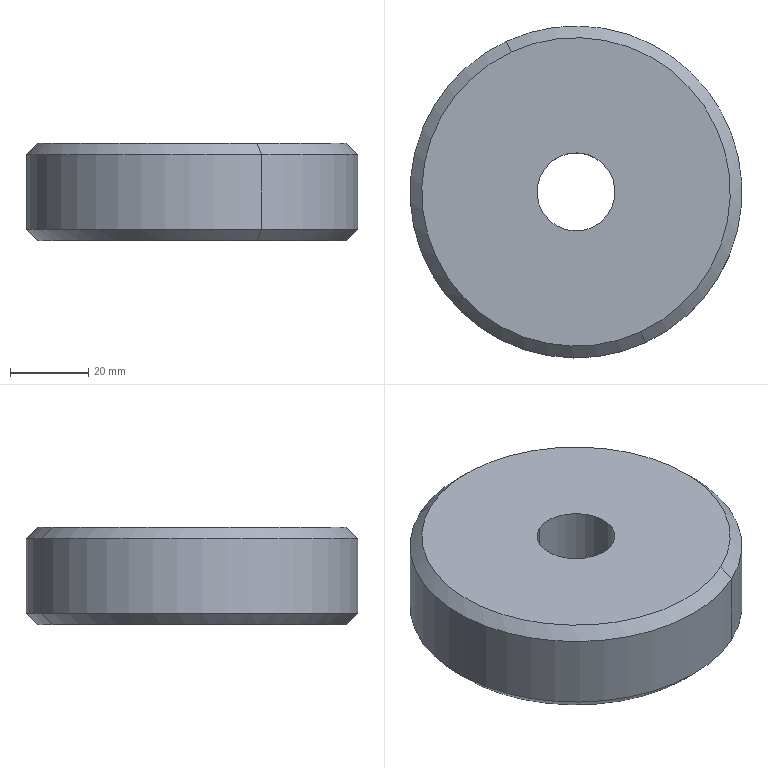Component | SolidWorks | Roller-10 | 1 solid | 10 faces | box 85 x 85 x 25 mm | volume 131662 mm3 | cone 4 | cylinder 4 | plane 2 | commonest cylinder face diameters 20 x2 85 x2 | material 45
build123d program:
from build123d import *

# Parameters (mm, degrees)
SKETCH1_R           = 42.5
SKETCH1_R_2         = 10
BOSS_EXTRUDE1_DEPTH = 25
CHAMFER1_SIZE       = 3


with BuildPart() as part:
    # Sketch1 → Boss-Extrude1 (new body)
    with BuildSketch(Plane.XY):
        with Locations((846.966, 841.557)):
            Circle(SKETCH1_R)
        with Locations((846.966, 841.557)):
            Circle(SKETCH1_R_2, mode=Mode.SUBTRACT)
    extrude(amount=BOSS_EXTRUDE1_DEPTH)

    # Chamfer1
    chamfer1_edges = [part.edges().sort_by_distance(p)[0] for p in [
        (804.466, 841.557, 0),
        (804.466, 841.557, 25),
    ]]
    chamfer(chamfer1_edges, length=CHAMFER1_SIZE)


solid = part.part

# Placed as in the assembly
solid = solid.moved(Location((103.122, -1001.49, 125), (0, 0, 0)))
STEP:
#1=CARTESIAN_POINT('',(38.059,-7.708,4.921));
#2=VERTEX_POINT('',#1);
#3=CARTESIAN_POINT('',(36.751,-4.886,4.921));
#4=VERTEX_POINT('',#3);
#5=CARTESIAN_POINT('',(37.405,-6.297,4.921));
#6=DIRECTION('',(0.,0.,-1.));
#7=DIRECTION('',(-0.4204,0.9074,0.));
#8=AXIS2_PLACEMENT_3D('',#5,#6,#7);
#9=CIRCLE('',#8,1.555);
#10=EDGE_CURVE('',#2,#4,#9,.T.);
#11=ORIENTED_EDGE('',*,*,#10,.F.);
#12=CARTESIAN_POINT('',(38.108,-7.815,5.039));
#13=VERTEX_POINT('',#12);
#14=CARTESIAN_POINT('',(38.108,-7.815,5.039));
#15=DIRECTION('',(0.2972,-0.6416,0.7071));
#16=VECTOR('',#15,39.37);
#17=LINE('',#14,#16);
#18=EDGE_CURVE('',#2,#13,#17,.T.);
#19=ORIENTED_EDGE('',*,*,#18,.T.);
#20=CARTESIAN_POINT('',(36.702,-4.778,5.039));
#21=VERTEX_POINT('',#20);
#22=CARTESIAN_POINT('',(37.405,-6.297,5.039));
#23=DIRECTION('',(-0.,-0.,1.));
#24=DIRECTION('',(-0.4204,0.9074,0.));
#25=AXIS2_PLACEMENT_3D('',#22,#23,#24);
#26=CIRCLE('',#25,1.673);
#27=EDGE_CURVE('',#21,#13,#26,.T.);
#28=ORIENTED_EDGE('',*,*,#27,.F.);
#29=CARTESIAN_POINT('',(36.702,-4.778,5.039));
#30=DIRECTION('',(-0.2972,0.6416,0.7071));
#31=VECTOR('',#30,39.37);
#32=LINE('',#29,#31);
#33=EDGE_CURVE('',#4,#21,#32,.T.);
#34=ORIENTED_EDGE('',*,*,#33,.F.);
#35=EDGE_LOOP('',(#11,#19,#28,#34));
#36=FACE_OUTER_BOUND('',#35,.T.);
#37=CARTESIAN_POINT('',(37.405,-6.297,5.039));
#38=DIRECTION('',(-0.,-0.,1.));
#39=DIRECTION('',(-0.4204,0.9074,0.));
#40=AXIS2_PLACEMENT_3D('',#37,#38,#39);
#41=CONICAL_SURFACE('',#40,1.673,0.7854);
#42=ADVANCED_FACE('',(#36),#41,.T.);
#43=CARTESIAN_POINT('',(36.751,-4.886,5.906));
#44=VERTEX_POINT('',#43);
#45=CARTESIAN_POINT('',(38.059,-7.708,5.906));
#46=VERTEX_POINT('',#45);
#47=CARTESIAN_POINT('',(37.405,-6.297,5.906));
#48=DIRECTION('',(-0.,-0.,1.));
#49=DIRECTION('',(-0.4204,0.9074,0.));
#50=AXIS2_PLACEMENT_3D('',#47,#48,#49);
#51=CIRCLE('',#50,1.555);
#52=EDGE_CURVE('',#44,#46,#51,.T.);
#53=ORIENTED_EDGE('',*,*,#52,.F.);
#54=CARTESIAN_POINT('',(36.702,-4.778,5.787));
#55=VERTEX_POINT('',#54);
#56=CARTESIAN_POINT('',(36.751,-4.886,5.906));
#57=DIRECTION('',(-0.2972,0.6416,-0.7071));
#58=VECTOR('',#57,39.37);
#59=LINE('',#56,#58);
#60=EDGE_CURVE('',#44,#55,#59,.T.);
#61=ORIENTED_EDGE('',*,*,#60,.T.);
#62=CARTESIAN_POINT('',(38.108,-7.815,5.787));
#63=VERTEX_POINT('',#62);
#64=CARTESIAN_POINT('',(37.405,-6.297,5.787));
#65=DIRECTION('',(0.,0.,-1.));
#66=DIRECTION('',(-0.4204,0.9074,0.));
#67=AXIS2_PLACEMENT_3D('',#64,#65,#66);
#68=CIRCLE('',#67,1.673);
#69=EDGE_CURVE('',#63,#55,#68,.T.);
#70=ORIENTED_EDGE('',*,*,#69,.F.);
#71=CARTESIAN_POINT('',(38.059,-7.708,5.906));
#72=DIRECTION('',(0.2972,-0.6416,-0.7071));
#73=VECTOR('',#72,39.37);
#74=LINE('',#71,#73);
#75=EDGE_CURVE('',#46,#63,#74,.T.);
#76=ORIENTED_EDGE('',*,*,#75,.F.);
#77=EDGE_LOOP('',(#53,#61,#70,#76));
#78=FACE_OUTER_BOUND('',#77,.T.);
#79=CARTESIAN_POINT('',(37.405,-6.297,5.906));
#80=DIRECTION('',(0.,0.,-1.));
#81=DIRECTION('',(0.4204,-0.9074,-0.));
#82=AXIS2_PLACEMENT_3D('',#79,#80,#81);
#83=CONICAL_SURFACE('',#82,1.555,0.7854);
#84=ADVANCED_FACE('',(#78),#83,.T.);
#85=CARTESIAN_POINT('',(37.571,-6.654,5.906));
#86=VERTEX_POINT('',#85);
#87=CARTESIAN_POINT('',(37.24,-5.939,5.906));
#88=VERTEX_POINT('',#87);
#89=CARTESIAN_POINT('',(37.405,-6.297,5.906));
#90=DIRECTION('',(-0.,-0.,1.));
#91=DIRECTION('',(-0.4204,0.9074,0.));
#92=AXIS2_PLACEMENT_3D('',#89,#90,#91);
#93=CIRCLE('',#92,0.3937);
#94=EDGE_CURVE('',#86,#88,#93,.T.);
#95=ORIENTED_EDGE('',*,*,#94,.T.);
#96=CARTESIAN_POINT('',(37.24,-5.939,4.921));
#97=VERTEX_POINT('',#96);
#98=CARTESIAN_POINT('',(37.24,-5.939,5.906));
#99=DIRECTION('',(0.,0.,-1.));
#100=VECTOR('',#99,39.37);
#101=LINE('',#98,#100);
#102=EDGE_CURVE('',#88,#97,#101,.T.);
#103=ORIENTED_EDGE('',*,*,#102,.T.);
#104=CARTESIAN_POINT('',(37.571,-6.654,4.921));
#105=VERTEX_POINT('',#104);
#106=CARTESIAN_POINT('',(37.405,-6.297,4.921));
#107=DIRECTION('',(-0.,-0.,1.));
#108=DIRECTION('',(-0.4204,0.9074,0.));
#109=AXIS2_PLACEMENT_3D('',#106,#107,#108);
#110=CIRCLE('',#109,0.3937);
#111=EDGE_CURVE('',#105,#97,#110,.T.);
#112=ORIENTED_EDGE('',*,*,#111,.F.);
#113=CARTESIAN_POINT('',(37.571,-6.654,5.906));
#114=DIRECTION('',(0.,0.,-1.));
#115=VECTOR('',#114,39.37);
#116=LINE('',#113,#115);
#117=EDGE_CURVE('',#86,#105,#116,.T.);
#118=ORIENTED_EDGE('',*,*,#117,.F.);
#119=EDGE_LOOP('',(#95,#103,#112,#118));
#120=FACE_OUTER_BOUND('',#119,.T.);
#121=CARTESIAN_POINT('',(37.405,-6.297,5.906));
#122=DIRECTION('',(0.,0.,-1.));
#123=DIRECTION('',(0.4204,-0.9074,0.));
#124=AXIS2_PLACEMENT_3D('',#121,#122,#123);
#125=CYLINDRICAL_SURFACE('',#124,0.3937);
#126=ADVANCED_FACE('',(#120),#125,.F.);
#127=ORIENTED_EDGE('',*,*,#69,.T.);
#128=CARTESIAN_POINT('',(36.702,-4.778,5.906));
#129=DIRECTION('',(0.,0.,-1.));
#130=VECTOR('',#129,39.37);
#131=LINE('',#128,#130);
#132=EDGE_CURVE('',#55,#21,#131,.T.);
#133=ORIENTED_EDGE('',*,*,#132,.T.);
#134=ORIENTED_EDGE('',*,*,#27,.T.);
#135=CARTESIAN_POINT('',(38.108,-7.815,5.906));
#136=DIRECTION('',(0.,0.,-1.));
#137=VECTOR('',#136,39.37);
#138=LINE('',#135,#137);
#139=EDGE_CURVE('',#63,#13,#138,.T.);
#140=ORIENTED_EDGE('',*,*,#139,.F.);
#141=EDGE_LOOP('',(#127,#133,#134,#140));
#142=FACE_OUTER_BOUND('',#141,.T.);
#143=CARTESIAN_POINT('',(37.405,-6.297,5.906));
#144=DIRECTION('',(0.,0.,-1.));
#145=DIRECTION('',(0.4204,-0.9074,-0.));
#146=AXIS2_PLACEMENT_3D('',#143,#144,#145);
#147=CYLINDRICAL_SURFACE('',#146,1.673);
#148=ADVANCED_FACE('',(#142),#147,.T.);
#149=CARTESIAN_POINT('',(37.405,-6.297,5.906));
#150=DIRECTION('',(-0.,-0.,1.));
#151=DIRECTION('',(-0.4204,0.9074,0.));
#152=AXIS2_PLACEMENT_3D('',#149,#150,#151);
#153=CIRCLE('',#152,1.555);
#154=EDGE_CURVE('',#46,#44,#153,.T.);
#155=ORIENTED_EDGE('',*,*,#154,.T.);
#156=ORIENTED_EDGE('',*,*,#52,.T.);
#157=EDGE_LOOP('',(#155,#156));
#158=FACE_OUTER_BOUND('',#157,.T.);
#159=ORIENTED_EDGE('',*,*,#94,.F.);
#160=CARTESIAN_POINT('',(37.405,-6.297,5.906));
#161=DIRECTION('',(-0.,-0.,1.));
#162=DIRECTION('',(-0.4204,0.9074,0.));
#163=AXIS2_PLACEMENT_3D('',#160,#161,#162);
#164=CIRCLE('',#163,0.3937);
#165=EDGE_CURVE('',#88,#86,#164,.T.);
#166=ORIENTED_EDGE('',*,*,#165,.F.);
#167=EDGE_LOOP('',(#159,#166));
#168=FACE_BOUND('',#167,.T.);
#169=CARTESIAN_POINT('',(37.405,-6.297,5.906));
#170=DIRECTION('',(-0.,-0.,1.));
#171=DIRECTION('',(-0.4204,0.9074,0.));
#172=AXIS2_PLACEMENT_3D('',#169,#170,#171);
#173=PLANE('',#172);
#174=ADVANCED_FACE('',(#158,#168),#173,.T.);
#175=CARTESIAN_POINT('',(37.405,-6.297,4.921));
#176=DIRECTION('',(0.,0.,-1.));
#177=DIRECTION('',(-0.4204,0.9074,0.));
#178=AXIS2_PLACEMENT_3D('',#175,#176,#177);
#179=CIRCLE('',#178,1.555);
#180=EDGE_CURVE('',#4,#2,#179,.T.);
#181=ORIENTED_EDGE('',*,*,#180,.T.);
#182=ORIENTED_EDGE('',*,*,#10,.T.);
#183=EDGE_LOOP('',(#181,#182));
#184=FACE_OUTER_BOUND('',#183,.T.);
#185=ORIENTED_EDGE('',*,*,#111,.T.);
#186=CARTESIAN_POINT('',(37.405,-6.297,4.921));
#187=DIRECTION('',(-0.,-0.,1.));
#188=DIRECTION('',(-0.4204,0.9074,0.));
#189=AXIS2_PLACEMENT_3D('',#186,#187,#188);
#190=CIRCLE('',#189,0.3937);
#191=EDGE_CURVE('',#97,#105,#190,.T.);
#192=ORIENTED_EDGE('',*,*,#191,.T.);
#193=EDGE_LOOP('',(#185,#192));
#194=FACE_BOUND('',#193,.T.);
#195=CARTESIAN_POINT('',(37.405,-6.297,4.921));
#196=DIRECTION('',(-0.,-0.,1.));
#197=DIRECTION('',(-0.4204,0.9074,0.));
#198=AXIS2_PLACEMENT_3D('',#195,#196,#197);
#199=PLANE('',#198);
#200=ADVANCED_FACE('',(#184,#194),#199,.F.);
#201=ORIENTED_EDGE('',*,*,#132,.F.);
#202=CARTESIAN_POINT('',(37.405,-6.297,5.787));
#203=DIRECTION('',(0.,0.,-1.));
#204=DIRECTION('',(-0.4204,0.9074,0.));
#205=AXIS2_PLACEMENT_3D('',#202,#203,#204);
#206=CIRCLE('',#205,1.673);
#207=EDGE_CURVE('',#55,#63,#206,.T.);
#208=ORIENTED_EDGE('',*,*,#207,.T.);
#209=ORIENTED_EDGE('',*,*,#139,.T.);
#210=CARTESIAN_POINT('',(37.405,-6.297,5.039));
#211=DIRECTION('',(-0.,-0.,1.));
#212=DIRECTION('',(-0.4204,0.9074,0.));
#213=AXIS2_PLACEMENT_3D('',#210,#211,#212);
#214=CIRCLE('',#213,1.673);
#215=EDGE_CURVE('',#13,#21,#214,.T.);
#216=ORIENTED_EDGE('',*,*,#215,.T.);
#217=EDGE_LOOP('',(#201,#208,#209,#216));
#218=FACE_OUTER_BOUND('',#217,.T.);
#219=CARTESIAN_POINT('',(37.405,-6.297,5.906));
#220=DIRECTION('',(0.,0.,-1.));
#221=DIRECTION('',(0.4204,-0.9074,-0.));
#222=AXIS2_PLACEMENT_3D('',#219,#220,#221);
#223=CYLINDRICAL_SURFACE('',#222,1.673);
#224=ADVANCED_FACE('',(#218),#223,.T.);
#225=ORIENTED_EDGE('',*,*,#102,.F.);
#226=ORIENTED_EDGE('',*,*,#165,.T.);
#227=ORIENTED_EDGE('',*,*,#117,.T.);
#228=ORIENTED_EDGE('',*,*,#191,.F.);
#229=EDGE_LOOP('',(#225,#226,#227,#228));
#230=FACE_OUTER_BOUND('',#229,.T.);
#231=CARTESIAN_POINT('',(37.405,-6.297,5.906));
#232=DIRECTION('',(0.,0.,-1.));
#233=DIRECTION('',(0.4204,-0.9074,0.));
#234=AXIS2_PLACEMENT_3D('',#231,#232,#233);
#235=CYLINDRICAL_SURFACE('',#234,0.3937);
#236=ADVANCED_FACE('',(#230),#235,.F.);
#237=ORIENTED_EDGE('',*,*,#60,.F.);
#238=ORIENTED_EDGE('',*,*,#154,.F.);
#239=ORIENTED_EDGE('',*,*,#75,.T.);
#240=ORIENTED_EDGE('',*,*,#207,.F.);
#241=EDGE_LOOP('',(#237,#238,#239,#240));
#242=FACE_OUTER_BOUND('',#241,.T.);
#243=CARTESIAN_POINT('',(37.405,-6.297,5.906));
#244=DIRECTION('',(0.,0.,-1.));
#245=DIRECTION('',(0.4204,-0.9074,-0.));
#246=AXIS2_PLACEMENT_3D('',#243,#244,#245);
#247=CONICAL_SURFACE('',#246,1.555,0.7854);
#248=ADVANCED_FACE('',(#242),#247,.T.);
#249=ORIENTED_EDGE('',*,*,#18,.F.);
#250=ORIENTED_EDGE('',*,*,#180,.F.);
#251=ORIENTED_EDGE('',*,*,#33,.T.);
#252=ORIENTED_EDGE('',*,*,#215,.F.);
#253=EDGE_LOOP('',(#249,#250,#251,#252));
#254=FACE_OUTER_BOUND('',#253,.T.);
#255=CARTESIAN_POINT('',(37.405,-6.297,5.039));
#256=DIRECTION('',(-0.,-0.,1.));
#257=DIRECTION('',(-0.4204,0.9074,0.));
#258=AXIS2_PLACEMENT_3D('',#255,#256,#257);
#259=CONICAL_SURFACE('',#258,1.673,0.7854);
#260=ADVANCED_FACE('',(#254),#259,.T.);
#261=CLOSED_SHELL('',(#42,#84,#126,#148,#174,#200,#224,#236,#248,#260));
#262=MANIFOLD_SOLID_BREP('',#261);
#263=CARTESIAN_POINT('',(0.,0.,0.));
#264=DIRECTION('',(0.,0.,1.));
#265=DIRECTION('',(1.,0.,0.));
#266=AXIS2_PLACEMENT_3D('',#263,#264,#265);
#267=(LENGTH_UNIT()NAMED_UNIT(*)SI_UNIT($,.METRE.));
#268=LENGTH_MEASURE_WITH_UNIT(LENGTH_MEASURE(0.0254),#267);
#269=DIMENSIONAL_EXPONENTS(1.,0.,0.,0.,0.,0.,0.);
#270=(CONVERSION_BASED_UNIT('',#268)LENGTH_UNIT()NAMED_UNIT(#269));
#271=UNCERTAINTY_MEASURE_WITH_UNIT(LENGTH_MEASURE(0.00001),#270,'','');
#272=(NAMED_UNIT(*)PLANE_ANGLE_UNIT()SI_UNIT($,.RADIAN.));
#273=(NAMED_UNIT(*)SI_UNIT($,.STERADIAN.)SOLID_ANGLE_UNIT());
#274=(GEOMETRIC_REPRESENTATION_CONTEXT(3)GLOBAL_UNCERTAINTY_ASSIGNED_CONTEXT((#271))GLOBAL_UNIT_ASSIGNED_CONTEXT((#270,#272,#273))REPRESENTATION_CONTEXT('',''));
#275=ADVANCED_BREP_SHAPE_REPRESENTATION('',(#262,#266),#274);
#276=COLOUR_RGB('',0.7922,0.8196,0.9333);
#277=FILL_AREA_STYLE_COLOUR('',#276);
#278=FILL_AREA_STYLE('',(#277));
#279=SURFACE_STYLE_FILL_AREA(#278);
#280=SURFACE_SIDE_STYLE('',(#279));
#281=SURFACE_STYLE_USAGE(.BOTH.,#280);
#282=PRESENTATION_STYLE_ASSIGNMENT((#281));
#283=STYLED_ITEM('',(#282),#262);
#284=PRESENTATION_LAYER_ASSIGNMENT('','',(#283));
#285=(LENGTH_UNIT()NAMED_UNIT(*)SI_UNIT($,.METRE.));
#286=LENGTH_MEASURE_WITH_UNIT(LENGTH_MEASURE(0.0254),#285);
#287=DIMENSIONAL_EXPONENTS(1.,0.,0.,0.,0.,0.,0.);
#288=(CONVERSION_BASED_UNIT('',#286)LENGTH_UNIT()NAMED_UNIT(#287));
#289=UNCERTAINTY_MEASURE_WITH_UNIT(LENGTH_MEASURE(0.00001),#288,'','');
#290=(NAMED_UNIT(*)PLANE_ANGLE_UNIT()SI_UNIT($,.RADIAN.));
#291=(NAMED_UNIT(*)SI_UNIT($,.STERADIAN.)SOLID_ANGLE_UNIT());
#292=(GEOMETRIC_REPRESENTATION_CONTEXT(3)GLOBAL_UNCERTAINTY_ASSIGNED_CONTEXT((#289))GLOBAL_UNIT_ASSIGNED_CONTEXT((#288,#290,#291))REPRESENTATION_CONTEXT('',''));
#293=MECHANICAL_DESIGN_GEOMETRIC_PRESENTATION_REPRESENTATION('',(#283),#292);